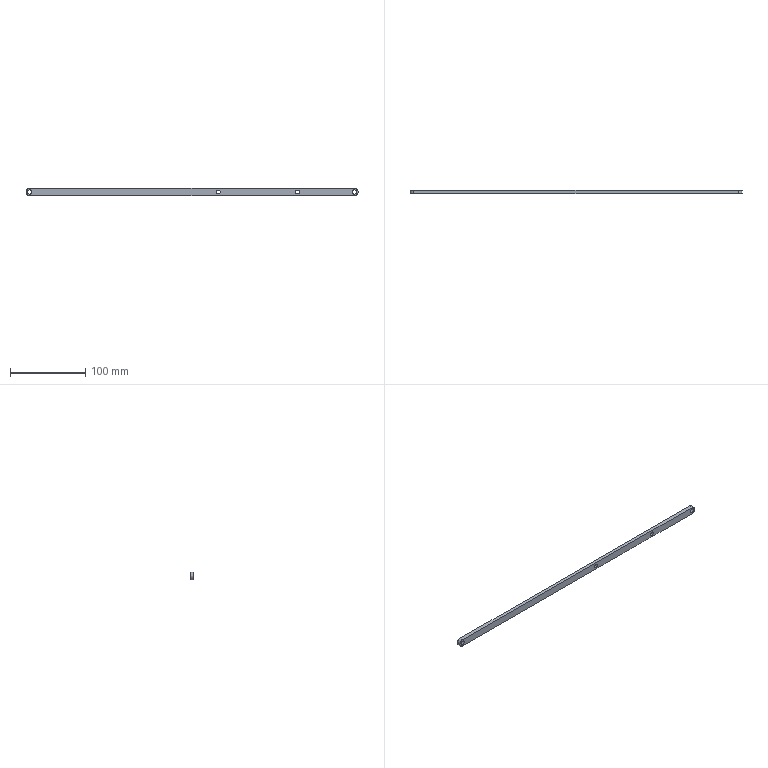Component | NX | 1 | 1 solid | 10 faces | box 440 x 5 x 10 mm | volume 21420 mm3 | cylinder 6 | plane 4 | commonest cylinder face diameters 10 x2 5 x2 5.929 x2
STEP:
#1=CARTESIAN_POINT('',(0.,0.,0.));
#2=DIRECTION('',(0.,0.,1.));
#3=DIRECTION('',(1.,0.,0.));
#4=AXIS2_PLACEMENT_3D('',#1,#2,#3);
#5=CARTESIAN_POINT('',(-501.588,50.95,5.));
#6=VERTEX_POINT('',#5);
#7=CARTESIAN_POINT('',(-71.588,50.95,5.));
#8=VERTEX_POINT('',#7);
#9=CARTESIAN_POINT('',(-501.588,50.95,5.));
#10=DIRECTION('',(1.,0.,-0.));
#11=VECTOR('',#10,1.);
#12=LINE('',#9,#11);
#13=CARTESIAN_POINT('',(-501.588,45.95,5.));
#14=DIRECTION('',(0.,0.,1.));
#15=DIRECTION('',(1.,0.,-0.));
#16=AXIS2_PLACEMENT_3D('',#13,#14,#15);
#17=PLANE('',#16);
#18=CARTESIAN_POINT('',(0.,5.));
#19=DIRECTION('',(1.,0.));
#20=VECTOR('',#19,1.);
#21=LINE('',#18,#20);
#22=(GEOMETRIC_REPRESENTATION_CONTEXT(2)PARAMETRIC_REPRESENTATION_CONTEXT()REPRESENTATION_CONTEXT('',''));
#23=DEFINITIONAL_REPRESENTATION('',(#21),#22);
#24=PCURVE('',#17,#23);
#25=CARTESIAN_POINT('',(-71.588,50.95,0.));
#26=DIRECTION('',(0.,1.,0.));
#27=DIRECTION('',(0.,0.,1.));
#28=AXIS2_PLACEMENT_3D('',#25,#26,#27);
#29=PLANE('',#28);
#30=CARTESIAN_POINT('',(5.,-430.));
#31=DIRECTION('',(-0.,1.));
#32=VECTOR('',#31,1.);
#33=LINE('',#30,#32);
#34=(GEOMETRIC_REPRESENTATION_CONTEXT(2)PARAMETRIC_REPRESENTATION_CONTEXT()REPRESENTATION_CONTEXT('',''));
#35=DEFINITIONAL_REPRESENTATION('',(#33),#34);
#36=PCURVE('',#29,#35);
#37=SURFACE_CURVE('',#12,(#24,#36),.PCURVE_S1.);
#38=EDGE_CURVE('',#6,#8,#37,.T.);
#39=ORIENTED_EDGE('',*,*,#38,.F.);
#40=CARTESIAN_POINT('',(-501.588,45.95,5.));
#41=VERTEX_POINT('',#40);
#42=CARTESIAN_POINT('',(-501.588,45.95,5.));
#43=DIRECTION('',(0.,1.,0.));
#44=VECTOR('',#43,1.);
#45=LINE('',#42,#44);
#46=CARTESIAN_POINT('',(0.,0.));
#47=DIRECTION('',(0.,1.));
#48=VECTOR('',#47,1.);
#49=LINE('',#46,#48);
#50=(GEOMETRIC_REPRESENTATION_CONTEXT(2)PARAMETRIC_REPRESENTATION_CONTEXT()REPRESENTATION_CONTEXT('',''));
#51=DEFINITIONAL_REPRESENTATION('',(#49),#50);
#52=PCURVE('',#17,#51);
#53=CARTESIAN_POINT('',(-501.588,45.95,0.));
#54=DIRECTION('',(0.,1.,0.));
#55=DIRECTION('',(0.,0.,1.));
#56=AXIS2_PLACEMENT_3D('',#53,#54,#55);
#57=CYLINDRICAL_SURFACE('',#56,5.);
#58=CARTESIAN_POINT('',(6.283,0.));
#59=DIRECTION('',(0.,1.));
#60=VECTOR('',#59,1.);
#61=LINE('',#58,#60);
#62=(GEOMETRIC_REPRESENTATION_CONTEXT(2)PARAMETRIC_REPRESENTATION_CONTEXT()REPRESENTATION_CONTEXT('',''));
#63=DEFINITIONAL_REPRESENTATION('',(#61),#62);
#64=PCURVE('',#57,#63);
#65=SURFACE_CURVE('',#45,(#52,#64),.PCURVE_S1.);
#66=EDGE_CURVE('',#41,#6,#65,.T.);
#67=ORIENTED_EDGE('',*,*,#66,.F.);
#68=CARTESIAN_POINT('',(-71.588,45.95,5.));
#69=VERTEX_POINT('',#68);
#70=CARTESIAN_POINT('',(-501.588,45.95,5.));
#71=DIRECTION('',(1.,0.,-0.));
#72=VECTOR('',#71,1.);
#73=LINE('',#70,#72);
#74=CARTESIAN_POINT('',(0.,0.));
#75=DIRECTION('',(1.,0.));
#76=VECTOR('',#75,1.);
#77=LINE('',#74,#76);
#78=(GEOMETRIC_REPRESENTATION_CONTEXT(2)PARAMETRIC_REPRESENTATION_CONTEXT()REPRESENTATION_CONTEXT('',''));
#79=DEFINITIONAL_REPRESENTATION('',(#77),#78);
#80=PCURVE('',#17,#79);
#81=CARTESIAN_POINT('',(-71.588,45.95,0.));
#82=DIRECTION('',(0.,1.,0.));
#83=DIRECTION('',(0.,0.,1.));
#84=AXIS2_PLACEMENT_3D('',#81,#82,#83);
#85=PLANE('',#84);
#86=CARTESIAN_POINT('',(5.,-430.));
#87=DIRECTION('',(-0.,1.));
#88=VECTOR('',#87,1.);
#89=LINE('',#86,#88);
#90=(GEOMETRIC_REPRESENTATION_CONTEXT(2)PARAMETRIC_REPRESENTATION_CONTEXT()REPRESENTATION_CONTEXT('',''));
#91=DEFINITIONAL_REPRESENTATION('',(#89),#90);
#92=PCURVE('',#85,#91);
#93=SURFACE_CURVE('',#73,(#80,#92),.PCURVE_S1.);
#94=EDGE_CURVE('',#41,#69,#93,.T.);
#95=ORIENTED_EDGE('',*,*,#94,.T.);
#96=CARTESIAN_POINT('',(-71.588,45.95,5.));
#97=DIRECTION('',(0.,1.,0.));
#98=VECTOR('',#97,1.);
#99=LINE('',#96,#98);
#100=CARTESIAN_POINT('',(430.,0.));
#101=DIRECTION('',(0.,1.));
#102=VECTOR('',#101,1.);
#103=LINE('',#100,#102);
#104=(GEOMETRIC_REPRESENTATION_CONTEXT(2)PARAMETRIC_REPRESENTATION_CONTEXT()REPRESENTATION_CONTEXT('',''));
#105=DEFINITIONAL_REPRESENTATION('',(#103),#104);
#106=PCURVE('',#17,#105);
#107=CARTESIAN_POINT('',(-71.588,45.95,0.));
#108=DIRECTION('',(0.,1.,0.));
#109=DIRECTION('',(0.,0.,1.));
#110=AXIS2_PLACEMENT_3D('',#107,#108,#109);
#111=CYLINDRICAL_SURFACE('',#110,5.);
#112=CARTESIAN_POINT('',(0.,0.));
#113=DIRECTION('',(0.,1.));
#114=VECTOR('',#113,1.);
#115=LINE('',#112,#114);
#116=(GEOMETRIC_REPRESENTATION_CONTEXT(2)PARAMETRIC_REPRESENTATION_CONTEXT()REPRESENTATION_CONTEXT('',''));
#117=DEFINITIONAL_REPRESENTATION('',(#115),#116);
#118=PCURVE('',#111,#117);
#119=SURFACE_CURVE('',#99,(#106,#118),.PCURVE_S1.);
#120=EDGE_CURVE('',#69,#8,#119,.T.);
#121=ORIENTED_EDGE('',*,*,#120,.T.);
#122=EDGE_LOOP('',(#39,#67,#95,#121));
#123=FACE_BOUND('',#122,.T.);
#124=ADVANCED_FACE('',(#123),#17,.T.);
#125=CARTESIAN_POINT('',(-71.588,50.95,-5.));
#126=VERTEX_POINT('',#125);
#127=CARTESIAN_POINT('',(-71.588,50.95,0.));
#128=DIRECTION('',(0.,1.,0.));
#129=DIRECTION('',(0.,0.,1.));
#130=AXIS2_PLACEMENT_3D('',#127,#128,#129);
#131=CIRCLE('',#130,5.);
#132=CARTESIAN_POINT('',(0.,5.));
#133=DIRECTION('',(1.,0.));
#134=VECTOR('',#133,1.);
#135=LINE('',#132,#134);
#136=(GEOMETRIC_REPRESENTATION_CONTEXT(2)PARAMETRIC_REPRESENTATION_CONTEXT()REPRESENTATION_CONTEXT('',''));
#137=DEFINITIONAL_REPRESENTATION('',(#135),#136);
#138=PCURVE('',#111,#137);
#139=CARTESIAN_POINT('',(0.,0.));
#140=DIRECTION('',(1.,0.));
#141=AXIS2_PLACEMENT_2D('',#139,#140);
#142=CIRCLE('',#141,5.);
#143=(GEOMETRIC_REPRESENTATION_CONTEXT(2)PARAMETRIC_REPRESENTATION_CONTEXT()REPRESENTATION_CONTEXT('',''));
#144=DEFINITIONAL_REPRESENTATION('',(#142),#143);
#145=PCURVE('',#29,#144);
#146=SURFACE_CURVE('',#131,(#138,#145),.PCURVE_S1.);
#147=EDGE_CURVE('',#8,#126,#146,.T.);
#148=ORIENTED_EDGE('',*,*,#147,.F.);
#149=ORIENTED_EDGE('',*,*,#120,.F.);
#150=CARTESIAN_POINT('',(-71.588,45.95,-5.));
#151=VERTEX_POINT('',#150);
#152=CARTESIAN_POINT('',(-71.588,45.95,0.));
#153=DIRECTION('',(0.,1.,0.));
#154=DIRECTION('',(0.,0.,1.));
#155=AXIS2_PLACEMENT_3D('',#152,#153,#154);
#156=CIRCLE('',#155,5.);
#157=CARTESIAN_POINT('',(0.,0.));
#158=DIRECTION('',(1.,0.));
#159=VECTOR('',#158,1.);
#160=LINE('',#157,#159);
#161=(GEOMETRIC_REPRESENTATION_CONTEXT(2)PARAMETRIC_REPRESENTATION_CONTEXT()REPRESENTATION_CONTEXT('',''));
#162=DEFINITIONAL_REPRESENTATION('',(#160),#161);
#163=PCURVE('',#111,#162);
#164=CARTESIAN_POINT('',(0.,0.));
#165=DIRECTION('',(1.,0.));
#166=AXIS2_PLACEMENT_2D('',#164,#165);
#167=CIRCLE('',#166,5.);
#168=(GEOMETRIC_REPRESENTATION_CONTEXT(2)PARAMETRIC_REPRESENTATION_CONTEXT()REPRESENTATION_CONTEXT('',''));
#169=DEFINITIONAL_REPRESENTATION('',(#167),#168);
#170=PCURVE('',#85,#169);
#171=SURFACE_CURVE('',#156,(#163,#170),.PCURVE_S1.);
#172=EDGE_CURVE('',#69,#151,#171,.T.);
#173=ORIENTED_EDGE('',*,*,#172,.T.);
#174=CARTESIAN_POINT('',(-71.588,45.95,-5.));
#175=DIRECTION('',(0.,1.,0.));
#176=VECTOR('',#175,1.);
#177=LINE('',#174,#176);
#178=CARTESIAN_POINT('',(3.142,0.));
#179=DIRECTION('',(0.,1.));
#180=VECTOR('',#179,1.);
#181=LINE('',#178,#180);
#182=(GEOMETRIC_REPRESENTATION_CONTEXT(2)PARAMETRIC_REPRESENTATION_CONTEXT()REPRESENTATION_CONTEXT('',''));
#183=DEFINITIONAL_REPRESENTATION('',(#181),#182);
#184=PCURVE('',#111,#183);
#185=CARTESIAN_POINT('',(-71.588,45.95,-5.));
#186=DIRECTION('',(0.,0.,-1.));
#187=DIRECTION('',(-1.,0.,-0.));
#188=AXIS2_PLACEMENT_3D('',#185,#186,#187);
#189=PLANE('',#188);
#190=CARTESIAN_POINT('',(0.,0.));
#191=DIRECTION('',(0.,1.));
#192=VECTOR('',#191,1.);
#193=LINE('',#190,#192);
#194=(GEOMETRIC_REPRESENTATION_CONTEXT(2)PARAMETRIC_REPRESENTATION_CONTEXT()REPRESENTATION_CONTEXT('',''));
#195=DEFINITIONAL_REPRESENTATION('',(#193),#194);
#196=PCURVE('',#189,#195);
#197=SURFACE_CURVE('',#177,(#184,#196),.PCURVE_S1.);
#198=EDGE_CURVE('',#151,#126,#197,.T.);
#199=ORIENTED_EDGE('',*,*,#198,.T.);
#200=EDGE_LOOP('',(#148,#149,#173,#199));
#201=FACE_BOUND('',#200,.T.);
#202=ADVANCED_FACE('',(#201),#111,.T.);
#203=CARTESIAN_POINT('',(-501.588,50.95,-5.));
#204=VERTEX_POINT('',#203);
#205=CARTESIAN_POINT('',(-71.588,50.95,-5.));
#206=DIRECTION('',(-1.,0.,-0.));
#207=VECTOR('',#206,1.);
#208=LINE('',#205,#207);
#209=CARTESIAN_POINT('',(0.,5.));
#210=DIRECTION('',(1.,0.));
#211=VECTOR('',#210,1.);
#212=LINE('',#209,#211);
#213=(GEOMETRIC_REPRESENTATION_CONTEXT(2)PARAMETRIC_REPRESENTATION_CONTEXT()REPRESENTATION_CONTEXT('',''));
#214=DEFINITIONAL_REPRESENTATION('',(#212),#213);
#215=PCURVE('',#189,#214);
#216=CARTESIAN_POINT('',(-5.,0.));
#217=DIRECTION('',(-0.,-1.));
#218=VECTOR('',#217,1.);
#219=LINE('',#216,#218);
#220=(GEOMETRIC_REPRESENTATION_CONTEXT(2)PARAMETRIC_REPRESENTATION_CONTEXT()REPRESENTATION_CONTEXT('',''));
#221=DEFINITIONAL_REPRESENTATION('',(#219),#220);
#222=PCURVE('',#29,#221);
#223=SURFACE_CURVE('',#208,(#215,#222),.PCURVE_S1.);
#224=EDGE_CURVE('',#126,#204,#223,.T.);
#225=ORIENTED_EDGE('',*,*,#224,.F.);
#226=ORIENTED_EDGE('',*,*,#198,.F.);
#227=CARTESIAN_POINT('',(-501.588,45.95,-5.));
#228=VERTEX_POINT('',#227);
#229=CARTESIAN_POINT('',(-71.588,45.95,-5.));
#230=DIRECTION('',(-1.,0.,-0.));
#231=VECTOR('',#230,1.);
#232=LINE('',#229,#231);
#233=CARTESIAN_POINT('',(0.,0.));
#234=DIRECTION('',(1.,0.));
#235=VECTOR('',#234,1.);
#236=LINE('',#233,#235);
#237=(GEOMETRIC_REPRESENTATION_CONTEXT(2)PARAMETRIC_REPRESENTATION_CONTEXT()REPRESENTATION_CONTEXT('',''));
#238=DEFINITIONAL_REPRESENTATION('',(#236),#237);
#239=PCURVE('',#189,#238);
#240=CARTESIAN_POINT('',(-5.,0.));
#241=DIRECTION('',(-0.,-1.));
#242=VECTOR('',#241,1.);
#243=LINE('',#240,#242);
#244=(GEOMETRIC_REPRESENTATION_CONTEXT(2)PARAMETRIC_REPRESENTATION_CONTEXT()REPRESENTATION_CONTEXT('',''));
#245=DEFINITIONAL_REPRESENTATION('',(#243),#244);
#246=PCURVE('',#85,#245);
#247=SURFACE_CURVE('',#232,(#239,#246),.PCURVE_S1.);
#248=EDGE_CURVE('',#151,#228,#247,.T.);
#249=ORIENTED_EDGE('',*,*,#248,.T.);
#250=CARTESIAN_POINT('',(-501.588,45.95,-5.));
#251=DIRECTION('',(0.,1.,0.));
#252=VECTOR('',#251,1.);
#253=LINE('',#250,#252);
#254=CARTESIAN_POINT('',(430.,0.));
#255=DIRECTION('',(0.,1.));
#256=VECTOR('',#255,1.);
#257=LINE('',#254,#256);
#258=(GEOMETRIC_REPRESENTATION_CONTEXT(2)PARAMETRIC_REPRESENTATION_CONTEXT()REPRESENTATION_CONTEXT('',''));
#259=DEFINITIONAL_REPRESENTATION('',(#257),#258);
#260=PCURVE('',#189,#259);
#261=CARTESIAN_POINT('',(3.142,0.));
#262=DIRECTION('',(0.,1.));
#263=VECTOR('',#262,1.);
#264=LINE('',#261,#263);
#265=(GEOMETRIC_REPRESENTATION_CONTEXT(2)PARAMETRIC_REPRESENTATION_CONTEXT()REPRESENTATION_CONTEXT('',''));
#266=DEFINITIONAL_REPRESENTATION('',(#264),#265);
#267=PCURVE('',#57,#266);
#268=SURFACE_CURVE('',#253,(#260,#267),.PCURVE_S1.);
#269=EDGE_CURVE('',#228,#204,#268,.T.);
#270=ORIENTED_EDGE('',*,*,#269,.T.);
#271=EDGE_LOOP('',(#225,#226,#249,#270));
#272=FACE_BOUND('',#271,.T.);
#273=ADVANCED_FACE('',(#272),#189,.T.);
#274=CARTESIAN_POINT('',(-251.588,45.95,2.5));
#275=VERTEX_POINT('',#274);
#276=CARTESIAN_POINT('',(-251.588,45.95,0.));
#277=DIRECTION('',(0.,-1.,0.));
#278=DIRECTION('',(0.,0.,1.));
#279=AXIS2_PLACEMENT_3D('',#276,#277,#278);
#280=CIRCLE('',#279,2.5);
#281=CARTESIAN_POINT('',(-251.588,45.95,0.));
#282=DIRECTION('',(0.,1.,0.));
#283=DIRECTION('',(0.,0.,1.));
#284=AXIS2_PLACEMENT_3D('',#281,#282,#283);
#285=CYLINDRICAL_SURFACE('',#284,2.5);
#286=CARTESIAN_POINT('',(6.283,0.));
#287=DIRECTION('',(-1.,0.));
#288=VECTOR('',#287,1.);
#289=LINE('',#286,#288);
#290=(GEOMETRIC_REPRESENTATION_CONTEXT(2)PARAMETRIC_REPRESENTATION_CONTEXT()REPRESENTATION_CONTEXT('',''));
#291=DEFINITIONAL_REPRESENTATION('',(#289),#290);
#292=PCURVE('',#285,#291);
#293=CARTESIAN_POINT('',(2.5,-180.));
#294=CARTESIAN_POINT('',(2.5,-184.33));
#295=CARTESIAN_POINT('',(-1.25,-182.165));
#296=CARTESIAN_POINT('',(-5.,-180.));
#297=CARTESIAN_POINT('',(-1.25,-177.835));
#298=CARTESIAN_POINT('',(2.5,-175.67));
#299=CARTESIAN_POINT('',(2.5,-180.));
#300=(BOUNDED_CURVE()B_SPLINE_CURVE(2,(#293,#294,#295,#296,#297,#298,#299),.UNSPECIFIED.,.T.,.F.)B_SPLINE_CURVE_WITH_KNOTS((1,2,2,2,2,1),(-2.094,0.,2.094,4.189,6.283,8.378),.UNSPECIFIED.)CURVE()GEOMETRIC_REPRESENTATION_ITEM()RATIONAL_B_SPLINE_CURVE((1.,0.5,1.,0.5,1.,0.5,1.))REPRESENTATION_ITEM(''));
#301=(GEOMETRIC_REPRESENTATION_CONTEXT(2)PARAMETRIC_REPRESENTATION_CONTEXT()REPRESENTATION_CONTEXT('',''));
#302=DEFINITIONAL_REPRESENTATION('',(#300),#301);
#303=PCURVE('',#85,#302);
#304=SURFACE_CURVE('',#280,(#292,#303),.PCURVE_S1.);
#305=EDGE_CURVE('',#275,#275,#304,.T.);
#306=ORIENTED_EDGE('',*,*,#305,.F.);
#307=CARTESIAN_POINT('',(-251.588,50.95,2.5));
#308=VERTEX_POINT('',#307);
#309=CARTESIAN_POINT('',(-251.588,45.95,2.5));
#310=CARTESIAN_POINT('',(-251.588,50.95,2.5));
#311=B_SPLINE_CURVE_WITH_KNOTS('',1,(#309,#310),.UNSPECIFIED.,.F.,.F.,(2,2),(0.,5.),.PIECEWISE_BEZIER_KNOTS.);
#312=CARTESIAN_POINT('',(6.283,0.));
#313=DIRECTION('',(0.,1.));
#314=VECTOR('',#313,1.);
#315=LINE('',#312,#314);
#316=(GEOMETRIC_REPRESENTATION_CONTEXT(2)PARAMETRIC_REPRESENTATION_CONTEXT()REPRESENTATION_CONTEXT('',''));
#317=DEFINITIONAL_REPRESENTATION('',(#315),#316);
#318=PCURVE('',#285,#317);
#319=CARTESIAN_POINT('',(0.,0.));
#320=DIRECTION('',(0.,1.));
#321=VECTOR('',#320,1.);
#322=LINE('',#319,#321);
#323=(GEOMETRIC_REPRESENTATION_CONTEXT(2)PARAMETRIC_REPRESENTATION_CONTEXT()REPRESENTATION_CONTEXT('',''));
#324=DEFINITIONAL_REPRESENTATION('',(#322),#323);
#325=PCURVE('',#285,#324);
#326=SEAM_CURVE('',#311,(#318,#325),.PCURVE_S1.);
#327=EDGE_CURVE('',#275,#308,#326,.T.);
#328=ORIENTED_EDGE('',*,*,#327,.T.);
#329=CARTESIAN_POINT('',(-251.588,50.95,0.));
#330=DIRECTION('',(0.,-1.,0.));
#331=DIRECTION('',(0.,0.,1.));
#332=AXIS2_PLACEMENT_3D('',#329,#330,#331);
#333=CIRCLE('',#332,2.5);
#334=CARTESIAN_POINT('',(6.283,5.));
#335=DIRECTION('',(-1.,0.));
#336=VECTOR('',#335,1.);
#337=LINE('',#334,#336);
#338=(GEOMETRIC_REPRESENTATION_CONTEXT(2)PARAMETRIC_REPRESENTATION_CONTEXT()REPRESENTATION_CONTEXT('',''));
#339=DEFINITIONAL_REPRESENTATION('',(#337),#338);
#340=PCURVE('',#285,#339);
#341=CARTESIAN_POINT('',(2.5,-180.));
#342=CARTESIAN_POINT('',(2.5,-184.33));
#343=CARTESIAN_POINT('',(-1.25,-182.165));
#344=CARTESIAN_POINT('',(-5.,-180.));
#345=CARTESIAN_POINT('',(-1.25,-177.835));
#346=CARTESIAN_POINT('',(2.5,-175.67));
#347=CARTESIAN_POINT('',(2.5,-180.));
#348=(BOUNDED_CURVE()B_SPLINE_CURVE(2,(#341,#342,#343,#344,#345,#346,#347),.UNSPECIFIED.,.T.,.F.)B_SPLINE_CURVE_WITH_KNOTS((1,2,2,2,2,1),(-2.094,0.,2.094,4.189,6.283,8.378),.UNSPECIFIED.)CURVE()GEOMETRIC_REPRESENTATION_ITEM()RATIONAL_B_SPLINE_CURVE((1.,0.5,1.,0.5,1.,0.5,1.))REPRESENTATION_ITEM(''));
#349=(GEOMETRIC_REPRESENTATION_CONTEXT(2)PARAMETRIC_REPRESENTATION_CONTEXT()REPRESENTATION_CONTEXT('',''));
#350=DEFINITIONAL_REPRESENTATION('',(#348),#349);
#351=PCURVE('',#29,#350);
#352=SURFACE_CURVE('',#333,(#340,#351),.PCURVE_S1.);
#353=EDGE_CURVE('',#308,#308,#352,.T.);
#354=ORIENTED_EDGE('',*,*,#353,.T.);
#355=ORIENTED_EDGE('',*,*,#327,.F.);
#356=EDGE_LOOP('',(#306,#328,#354,#355));
#357=FACE_BOUND('',#356,.F.);
#358=ADVANCED_FACE('',(#357),#285,.F.);
#359=CARTESIAN_POINT('',(-501.588,45.95,2.964));
#360=VERTEX_POINT('',#359);
#361=CARTESIAN_POINT('',(-501.588,45.95,0.));
#362=DIRECTION('',(0.,1.,0.));
#363=DIRECTION('',(0.,0.,1.));
#364=AXIS2_PLACEMENT_3D('',#361,#362,#363);
#365=CIRCLE('',#364,2.964);
#366=CARTESIAN_POINT('',(-501.588,45.95,0.));
#367=DIRECTION('',(0.,1.,0.));
#368=DIRECTION('',(0.,0.,1.));
#369=AXIS2_PLACEMENT_3D('',#366,#367,#368);
#370=CYLINDRICAL_SURFACE('',#369,2.964);
#371=CARTESIAN_POINT('',(0.,0.));
#372=DIRECTION('',(1.,0.));
#373=VECTOR('',#372,1.);
#374=LINE('',#371,#373);
#375=(GEOMETRIC_REPRESENTATION_CONTEXT(2)PARAMETRIC_REPRESENTATION_CONTEXT()REPRESENTATION_CONTEXT('',''));
#376=DEFINITIONAL_REPRESENTATION('',(#374),#375);
#377=PCURVE('',#370,#376);
#378=CARTESIAN_POINT('',(0.,-430.));
#379=DIRECTION('',(1.,0.));
#380=AXIS2_PLACEMENT_2D('',#378,#379);
#381=CIRCLE('',#380,2.964);
#382=(GEOMETRIC_REPRESENTATION_CONTEXT(2)PARAMETRIC_REPRESENTATION_CONTEXT()REPRESENTATION_CONTEXT('',''));
#383=DEFINITIONAL_REPRESENTATION('',(#381),#382);
#384=PCURVE('',#85,#383);
#385=SURFACE_CURVE('',#365,(#377,#384),.PCURVE_S1.);
#386=EDGE_CURVE('',#360,#360,#385,.T.);
#387=ORIENTED_EDGE('',*,*,#386,.T.);
#388=CARTESIAN_POINT('',(-501.588,50.95,2.964));
#389=VERTEX_POINT('',#388);
#390=CARTESIAN_POINT('',(-501.588,45.95,2.964));
#391=CARTESIAN_POINT('',(-501.588,50.95,2.964));
#392=B_SPLINE_CURVE_WITH_KNOTS('',1,(#390,#391),.UNSPECIFIED.,.F.,.F.,(2,2),(0.,5.),.PIECEWISE_BEZIER_KNOTS.);
#393=CARTESIAN_POINT('',(6.283,0.));
#394=DIRECTION('',(0.,1.));
#395=VECTOR('',#394,1.);
#396=LINE('',#393,#395);
#397=(GEOMETRIC_REPRESENTATION_CONTEXT(2)PARAMETRIC_REPRESENTATION_CONTEXT()REPRESENTATION_CONTEXT('',''));
#398=DEFINITIONAL_REPRESENTATION('',(#396),#397);
#399=PCURVE('',#370,#398);
#400=CARTESIAN_POINT('',(0.,0.));
#401=DIRECTION('',(0.,1.));
#402=VECTOR('',#401,1.);
#403=LINE('',#400,#402);
#404=(GEOMETRIC_REPRESENTATION_CONTEXT(2)PARAMETRIC_REPRESENTATION_CONTEXT()REPRESENTATION_CONTEXT('',''));
#405=DEFINITIONAL_REPRESENTATION('',(#403),#404);
#406=PCURVE('',#370,#405);
#407=SEAM_CURVE('',#392,(#399,#406),.PCURVE_S1.);
#408=EDGE_CURVE('',#360,#389,#407,.T.);
#409=ORIENTED_EDGE('',*,*,#408,.T.);
#410=CARTESIAN_POINT('',(-501.588,50.95,0.));
#411=DIRECTION('',(0.,1.,0.));
#412=DIRECTION('',(0.,0.,1.));
#413=AXIS2_PLACEMENT_3D('',#410,#411,#412);
#414=CIRCLE('',#413,2.964);
#415=CARTESIAN_POINT('',(0.,5.));
#416=DIRECTION('',(1.,0.));
#417=VECTOR('',#416,1.);
#418=LINE('',#415,#417);
#419=(GEOMETRIC_REPRESENTATION_CONTEXT(2)PARAMETRIC_REPRESENTATION_CONTEXT()REPRESENTATION_CONTEXT('',''));
#420=DEFINITIONAL_REPRESENTATION('',(#418),#419);
#421=PCURVE('',#370,#420);
#422=CARTESIAN_POINT('',(0.,-430.));
#423=DIRECTION('',(1.,0.));
#424=AXIS2_PLACEMENT_2D('',#422,#423);
#425=CIRCLE('',#424,2.964);
#426=(GEOMETRIC_REPRESENTATION_CONTEXT(2)PARAMETRIC_REPRESENTATION_CONTEXT()REPRESENTATION_CONTEXT('',''));
#427=DEFINITIONAL_REPRESENTATION('',(#425),#426);
#428=PCURVE('',#29,#427);
#429=SURFACE_CURVE('',#414,(#421,#428),.PCURVE_S1.);
#430=EDGE_CURVE('',#389,#389,#429,.T.);
#431=ORIENTED_EDGE('',*,*,#430,.F.);
#432=ORIENTED_EDGE('',*,*,#408,.F.);
#433=EDGE_LOOP('',(#387,#409,#431,#432));
#434=FACE_BOUND('',#433,.F.);
#435=ADVANCED_FACE('',(#434),#370,.F.);
#436=CARTESIAN_POINT('',(-146.793,45.95,2.5));
#437=VERTEX_POINT('',#436);
#438=CARTESIAN_POINT('',(-146.793,45.95,0.));
#439=DIRECTION('',(0.,-1.,0.));
#440=DIRECTION('',(0.,0.,1.));
#441=AXIS2_PLACEMENT_3D('',#438,#439,#440);
#442=CIRCLE('',#441,2.5);
#443=CARTESIAN_POINT('',(-146.793,45.95,0.));
#444=DIRECTION('',(0.,1.,0.));
#445=DIRECTION('',(0.,0.,1.));
#446=AXIS2_PLACEMENT_3D('',#443,#444,#445);
#447=CYLINDRICAL_SURFACE('',#446,2.5);
#448=CARTESIAN_POINT('',(6.283,0.));
#449=DIRECTION('',(-1.,0.));
#450=VECTOR('',#449,1.);
#451=LINE('',#448,#450);
#452=(GEOMETRIC_REPRESENTATION_CONTEXT(2)PARAMETRIC_REPRESENTATION_CONTEXT()REPRESENTATION_CONTEXT('',''));
#453=DEFINITIONAL_REPRESENTATION('',(#451),#452);
#454=PCURVE('',#447,#453);
#455=CARTESIAN_POINT('',(2.5,-75.206));
#456=CARTESIAN_POINT('',(2.5,-79.536));
#457=CARTESIAN_POINT('',(-1.25,-77.371));
#458=CARTESIAN_POINT('',(-5.,-75.206));
#459=CARTESIAN_POINT('',(-1.25,-73.04));
#460=CARTESIAN_POINT('',(2.5,-70.875));
#461=CARTESIAN_POINT('',(2.5,-75.206));
#462=(BOUNDED_CURVE()B_SPLINE_CURVE(2,(#455,#456,#457,#458,#459,#460,#461),.UNSPECIFIED.,.T.,.F.)B_SPLINE_CURVE_WITH_KNOTS((1,2,2,2,2,1),(-2.094,0.,2.094,4.189,6.283,8.378),.UNSPECIFIED.)CURVE()GEOMETRIC_REPRESENTATION_ITEM()RATIONAL_B_SPLINE_CURVE((1.,0.5,1.,0.5,1.,0.5,1.))REPRESENTATION_ITEM(''));
#463=(GEOMETRIC_REPRESENTATION_CONTEXT(2)PARAMETRIC_REPRESENTATION_CONTEXT()REPRESENTATION_CONTEXT('',''));
#464=DEFINITIONAL_REPRESENTATION('',(#462),#463);
#465=PCURVE('',#85,#464);
#466=SURFACE_CURVE('',#442,(#454,#465),.PCURVE_S1.);
#467=EDGE_CURVE('',#437,#437,#466,.T.);
#468=ORIENTED_EDGE('',*,*,#467,.F.);
#469=CARTESIAN_POINT('',(-146.793,50.95,2.5));
#470=VERTEX_POINT('',#469);
#471=CARTESIAN_POINT('',(-146.793,45.95,2.5));
#472=CARTESIAN_POINT('',(-146.793,50.95,2.5));
#473=B_SPLINE_CURVE_WITH_KNOTS('',1,(#471,#472),.UNSPECIFIED.,.F.,.F.,(2,2),(0.,5.),.PIECEWISE_BEZIER_KNOTS.);
#474=CARTESIAN_POINT('',(6.283,0.));
#475=DIRECTION('',(0.,1.));
#476=VECTOR('',#475,1.);
#477=LINE('',#474,#476);
#478=(GEOMETRIC_REPRESENTATION_CONTEXT(2)PARAMETRIC_REPRESENTATION_CONTEXT()REPRESENTATION_CONTEXT('',''));
#479=DEFINITIONAL_REPRESENTATION('',(#477),#478);
#480=PCURVE('',#447,#479);
#481=CARTESIAN_POINT('',(0.,0.));
#482=DIRECTION('',(0.,1.));
#483=VECTOR('',#482,1.);
#484=LINE('',#481,#483);
#485=(GEOMETRIC_REPRESENTATION_CONTEXT(2)PARAMETRIC_REPRESENTATION_CONTEXT()REPRESENTATION_CONTEXT('',''));
#486=DEFINITIONAL_REPRESENTATION('',(#484),#485);
#487=PCURVE('',#447,#486);
#488=SEAM_CURVE('',#473,(#480,#487),.PCURVE_S1.);
#489=EDGE_CURVE('',#437,#470,#488,.T.);
#490=ORIENTED_EDGE('',*,*,#489,.T.);
#491=CARTESIAN_POINT('',(-146.793,50.95,0.));
#492=DIRECTION('',(0.,-1.,0.));
#493=DIRECTION('',(0.,0.,1.));
#494=AXIS2_PLACEMENT_3D('',#491,#492,#493);
#495=CIRCLE('',#494,2.5);
#496=CARTESIAN_POINT('',(6.283,5.));
#497=DIRECTION('',(-1.,0.));
#498=VECTOR('',#497,1.);
#499=LINE('',#496,#498);
#500=(GEOMETRIC_REPRESENTATION_CONTEXT(2)PARAMETRIC_REPRESENTATION_CONTEXT()REPRESENTATION_CONTEXT('',''));
#501=DEFINITIONAL_REPRESENTATION('',(#499),#500);
#502=PCURVE('',#447,#501);
#503=CARTESIAN_POINT('',(2.5,-75.206));
#504=CARTESIAN_POINT('',(2.5,-79.536));
#505=CARTESIAN_POINT('',(-1.25,-77.371));
#506=CARTESIAN_POINT('',(-5.,-75.206));
#507=CARTESIAN_POINT('',(-1.25,-73.04));
#508=CARTESIAN_POINT('',(2.5,-70.875));
#509=CARTESIAN_POINT('',(2.5,-75.206));
#510=(BOUNDED_CURVE()B_SPLINE_CURVE(2,(#503,#504,#505,#506,#507,#508,#509),.UNSPECIFIED.,.T.,.F.)B_SPLINE_CURVE_WITH_KNOTS((1,2,2,2,2,1),(-2.094,0.,2.094,4.189,6.283,8.378),.UNSPECIFIED.)CURVE()GEOMETRIC_REPRESENTATION_ITEM()RATIONAL_B_SPLINE_CURVE((1.,0.5,1.,0.5,1.,0.5,1.))REPRESENTATION_ITEM(''));
#511=(GEOMETRIC_REPRESENTATION_CONTEXT(2)PARAMETRIC_REPRESENTATION_CONTEXT()REPRESENTATION_CONTEXT('',''));
#512=DEFINITIONAL_REPRESENTATION('',(#510),#511);
#513=PCURVE('',#29,#512);
#514=SURFACE_CURVE('',#495,(#502,#513),.PCURVE_S1.);
#515=EDGE_CURVE('',#470,#470,#514,.T.);
#516=ORIENTED_EDGE('',*,*,#515,.T.);
#517=ORIENTED_EDGE('',*,*,#489,.F.);
#518=EDGE_LOOP('',(#468,#490,#516,#517));
#519=FACE_BOUND('',#518,.F.);
#520=ADVANCED_FACE('',(#519),#447,.F.);
#521=CARTESIAN_POINT('',(-501.588,50.95,0.));
#522=DIRECTION('',(0.,1.,0.));
#523=DIRECTION('',(0.,0.,1.));
#524=AXIS2_PLACEMENT_3D('',#521,#522,#523);
#525=CIRCLE('',#524,5.);
#526=CARTESIAN_POINT('',(0.,5.));
#527=DIRECTION('',(1.,0.));
#528=VECTOR('',#527,1.);
#529=LINE('',#526,#528);
#530=(GEOMETRIC_REPRESENTATION_CONTEXT(2)PARAMETRIC_REPRESENTATION_CONTEXT()REPRESENTATION_CONTEXT('',''));
#531=DEFINITIONAL_REPRESENTATION('',(#529),#530);
#532=PCURVE('',#57,#531);
#533=CARTESIAN_POINT('',(0.,-430.));
#534=DIRECTION('',(1.,0.));
#535=AXIS2_PLACEMENT_2D('',#533,#534);
#536=CIRCLE('',#535,5.);
#537=(GEOMETRIC_REPRESENTATION_CONTEXT(2)PARAMETRIC_REPRESENTATION_CONTEXT()REPRESENTATION_CONTEXT('',''));
#538=DEFINITIONAL_REPRESENTATION('',(#536),#537);
#539=PCURVE('',#29,#538);
#540=SURFACE_CURVE('',#525,(#532,#539),.PCURVE_S1.);
#541=EDGE_CURVE('',#204,#6,#540,.T.);
#542=ORIENTED_EDGE('',*,*,#541,.F.);
#543=ORIENTED_EDGE('',*,*,#269,.F.);
#544=CARTESIAN_POINT('',(-501.588,45.95,0.));
#545=DIRECTION('',(0.,1.,0.));
#546=DIRECTION('',(0.,0.,1.));
#547=AXIS2_PLACEMENT_3D('',#544,#545,#546);
#548=CIRCLE('',#547,5.);
#549=CARTESIAN_POINT('',(0.,0.));
#550=DIRECTION('',(1.,0.));
#551=VECTOR('',#550,1.);
#552=LINE('',#549,#551);
#553=(GEOMETRIC_REPRESENTATION_CONTEXT(2)PARAMETRIC_REPRESENTATION_CONTEXT()REPRESENTATION_CONTEXT('',''));
#554=DEFINITIONAL_REPRESENTATION('',(#552),#553);
#555=PCURVE('',#57,#554);
#556=CARTESIAN_POINT('',(0.,-430.));
#557=DIRECTION('',(1.,0.));
#558=AXIS2_PLACEMENT_2D('',#556,#557);
#559=CIRCLE('',#558,5.);
#560=(GEOMETRIC_REPRESENTATION_CONTEXT(2)PARAMETRIC_REPRESENTATION_CONTEXT()REPRESENTATION_CONTEXT('',''));
#561=DEFINITIONAL_REPRESENTATION('',(#559),#560);
#562=PCURVE('',#85,#561);
#563=SURFACE_CURVE('',#548,(#555,#562),.PCURVE_S1.);
#564=EDGE_CURVE('',#228,#41,#563,.T.);
#565=ORIENTED_EDGE('',*,*,#564,.T.);
#566=ORIENTED_EDGE('',*,*,#66,.T.);
#567=EDGE_LOOP('',(#542,#543,#565,#566));
#568=FACE_BOUND('',#567,.T.);
#569=ADVANCED_FACE('',(#568),#57,.T.);
#570=CARTESIAN_POINT('',(-71.588,45.95,2.964));
#571=VERTEX_POINT('',#570);
#572=CARTESIAN_POINT('',(-71.588,45.95,0.));
#573=DIRECTION('',(0.,1.,0.));
#574=DIRECTION('',(0.,0.,1.));
#575=AXIS2_PLACEMENT_3D('',#572,#573,#574);
#576=CIRCLE('',#575,2.964);
#577=CARTESIAN_POINT('',(-71.588,45.95,0.));
#578=DIRECTION('',(0.,1.,0.));
#579=DIRECTION('',(0.,0.,1.));
#580=AXIS2_PLACEMENT_3D('',#577,#578,#579);
#581=CYLINDRICAL_SURFACE('',#580,2.964);
#582=CARTESIAN_POINT('',(0.,0.));
#583=DIRECTION('',(1.,0.));
#584=VECTOR('',#583,1.);
#585=LINE('',#582,#584);
#586=(GEOMETRIC_REPRESENTATION_CONTEXT(2)PARAMETRIC_REPRESENTATION_CONTEXT()REPRESENTATION_CONTEXT('',''));
#587=DEFINITIONAL_REPRESENTATION('',(#585),#586);
#588=PCURVE('',#581,#587);
#589=CARTESIAN_POINT('',(0.,0.));
#590=DIRECTION('',(1.,0.));
#591=AXIS2_PLACEMENT_2D('',#589,#590);
#592=CIRCLE('',#591,2.964);
#593=(GEOMETRIC_REPRESENTATION_CONTEXT(2)PARAMETRIC_REPRESENTATION_CONTEXT()REPRESENTATION_CONTEXT('',''));
#594=DEFINITIONAL_REPRESENTATION('',(#592),#593);
#595=PCURVE('',#85,#594);
#596=SURFACE_CURVE('',#576,(#588,#595),.PCURVE_S1.);
#597=EDGE_CURVE('',#571,#571,#596,.T.);
#598=ORIENTED_EDGE('',*,*,#597,.T.);
#599=CARTESIAN_POINT('',(-71.588,50.95,2.964));
#600=VERTEX_POINT('',#599);
#601=CARTESIAN_POINT('',(-71.588,45.95,2.964));
#602=CARTESIAN_POINT('',(-71.588,50.95,2.964));
#603=B_SPLINE_CURVE_WITH_KNOTS('',1,(#601,#602),.UNSPECIFIED.,.F.,.F.,(2,2),(0.,5.),.PIECEWISE_BEZIER_KNOTS.);
#604=CARTESIAN_POINT('',(6.283,0.));
#605=DIRECTION('',(0.,1.));
#606=VECTOR('',#605,1.);
#607=LINE('',#604,#606);
#608=(GEOMETRIC_REPRESENTATION_CONTEXT(2)PARAMETRIC_REPRESENTATION_CONTEXT()REPRESENTATION_CONTEXT('',''));
#609=DEFINITIONAL_REPRESENTATION('',(#607),#608);
#610=PCURVE('',#581,#609);
#611=CARTESIAN_POINT('',(0.,0.));
#612=DIRECTION('',(0.,1.));
#613=VECTOR('',#612,1.);
#614=LINE('',#611,#613);
#615=(GEOMETRIC_REPRESENTATION_CONTEXT(2)PARAMETRIC_REPRESENTATION_CONTEXT()REPRESENTATION_CONTEXT('',''));
#616=DEFINITIONAL_REPRESENTATION('',(#614),#615);
#617=PCURVE('',#581,#616);
#618=SEAM_CURVE('',#603,(#610,#617),.PCURVE_S1.);
#619=EDGE_CURVE('',#571,#600,#618,.T.);
#620=ORIENTED_EDGE('',*,*,#619,.T.);
#621=CARTESIAN_POINT('',(-71.588,50.95,0.));
#622=DIRECTION('',(0.,1.,0.));
#623=DIRECTION('',(0.,0.,1.));
#624=AXIS2_PLACEMENT_3D('',#621,#622,#623);
#625=CIRCLE('',#624,2.964);
#626=CARTESIAN_POINT('',(0.,5.));
#627=DIRECTION('',(1.,0.));
#628=VECTOR('',#627,1.);
#629=LINE('',#626,#628);
#630=(GEOMETRIC_REPRESENTATION_CONTEXT(2)PARAMETRIC_REPRESENTATION_CONTEXT()REPRESENTATION_CONTEXT('',''));
#631=DEFINITIONAL_REPRESENTATION('',(#629),#630);
#632=PCURVE('',#581,#631);
#633=CARTESIAN_POINT('',(0.,0.));
#634=DIRECTION('',(1.,0.));
#635=AXIS2_PLACEMENT_2D('',#633,#634);
#636=CIRCLE('',#635,2.964);
#637=(GEOMETRIC_REPRESENTATION_CONTEXT(2)PARAMETRIC_REPRESENTATION_CONTEXT()REPRESENTATION_CONTEXT('',''));
#638=DEFINITIONAL_REPRESENTATION('',(#636),#637);
#639=PCURVE('',#29,#638);
#640=SURFACE_CURVE('',#625,(#632,#639),.PCURVE_S1.);
#641=EDGE_CURVE('',#600,#600,#640,.T.);
#642=ORIENTED_EDGE('',*,*,#641,.F.);
#643=ORIENTED_EDGE('',*,*,#619,.F.);
#644=EDGE_LOOP('',(#598,#620,#642,#643));
#645=FACE_BOUND('',#644,.F.);
#646=ADVANCED_FACE('',(#645),#581,.F.);
#647=ORIENTED_EDGE('',*,*,#94,.F.);
#648=ORIENTED_EDGE('',*,*,#564,.F.);
#649=ORIENTED_EDGE('',*,*,#248,.F.);
#650=ORIENTED_EDGE('',*,*,#172,.F.);
#651=EDGE_LOOP('',(#647,#648,#649,#650));
#652=FACE_BOUND('',#651,.T.);
#653=ORIENTED_EDGE('',*,*,#467,.F.);
#654=EDGE_LOOP('',(#653));
#655=FACE_BOUND('',#654,.T.);
#656=ORIENTED_EDGE('',*,*,#386,.T.);
#657=EDGE_LOOP('',(#656));
#658=FACE_BOUND('',#657,.T.);
#659=ORIENTED_EDGE('',*,*,#305,.F.);
#660=EDGE_LOOP('',(#659));
#661=FACE_BOUND('',#660,.T.);
#662=ORIENTED_EDGE('',*,*,#597,.T.);
#663=EDGE_LOOP('',(#662));
#664=FACE_BOUND('',#663,.T.);
#665=ADVANCED_FACE('',(#652,#655,#658,#661,#664),#85,.F.);
#666=ORIENTED_EDGE('',*,*,#38,.T.);
#667=ORIENTED_EDGE('',*,*,#147,.T.);
#668=ORIENTED_EDGE('',*,*,#224,.T.);
#669=ORIENTED_EDGE('',*,*,#541,.T.);
#670=EDGE_LOOP('',(#666,#667,#668,#669));
#671=FACE_BOUND('',#670,.T.);
#672=ORIENTED_EDGE('',*,*,#515,.T.);
#673=EDGE_LOOP('',(#672));
#674=FACE_BOUND('',#673,.T.);
#675=ORIENTED_EDGE('',*,*,#430,.F.);
#676=EDGE_LOOP('',(#675));
#677=FACE_BOUND('',#676,.T.);
#678=ORIENTED_EDGE('',*,*,#353,.T.);
#679=EDGE_LOOP('',(#678));
#680=FACE_BOUND('',#679,.T.);
#681=ORIENTED_EDGE('',*,*,#641,.F.);
#682=EDGE_LOOP('',(#681));
#683=FACE_BOUND('',#682,.T.);
#684=ADVANCED_FACE('',(#671,#674,#677,#680,#683),#29,.T.);
#685=CLOSED_SHELL('',(#124,#202,#273,#358,#435,#520,#569,#646,#665,#684));
#686=MANIFOLD_SOLID_BREP('',#685);
#687=(LENGTH_UNIT()NAMED_UNIT(*)SI_UNIT(.MILLI.,.METRE.));
#688=UNCERTAINTY_MEASURE_WITH_UNIT(LENGTH_MEASURE(0.000005),#687,'','');
#689=(NAMED_UNIT(*)PLANE_ANGLE_UNIT()SI_UNIT($,.RADIAN.));
#690=(NAMED_UNIT(*)SI_UNIT($,.STERADIAN.)SOLID_ANGLE_UNIT());
#691=(GEOMETRIC_REPRESENTATION_CONTEXT(3)GLOBAL_UNCERTAINTY_ASSIGNED_CONTEXT((#688))GLOBAL_UNIT_ASSIGNED_CONTEXT((#687,#689,#690))REPRESENTATION_CONTEXT('',''));
#692=ADVANCED_BREP_SHAPE_REPRESENTATION('',(#4,#686),#691);